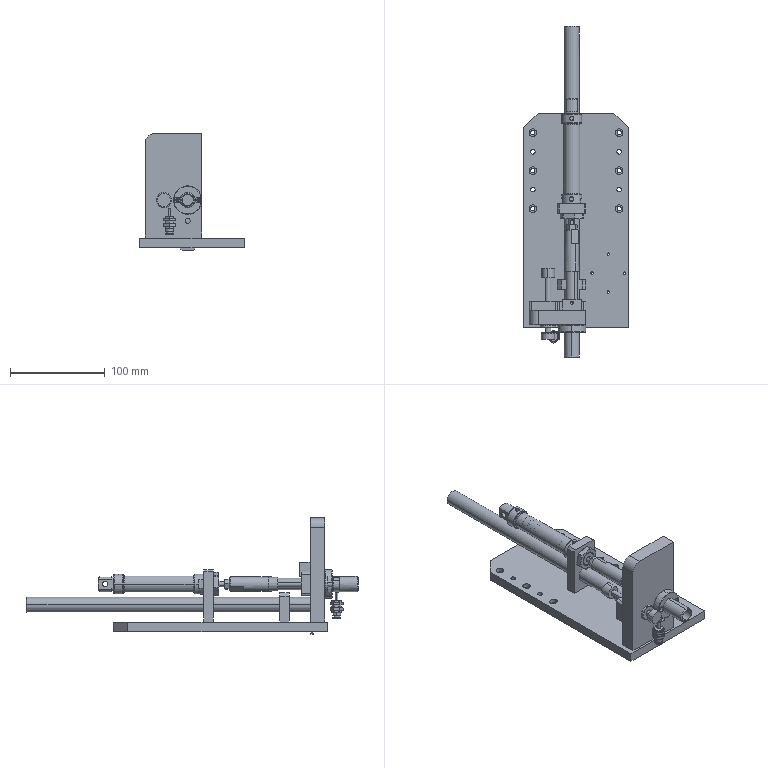Assembly | SolidWorks | mm | 21 component files | 21 solids | 613 faces | box 110 x 349.9 x 123 mm | volume 442250 mm3 | cylinder 275 | plane 190 | cone 140 | spline 8 | commonest cylinder face diameters 6 x30 8 x30 4.5 x30 3.3 x26 12 x17 5 x16 2.5 x16 16 x14
Bill of materials:
gbgb16 MA NutF8 | 1 |  | Thin, flat hexagonal ring with a large central through-bore. One face is chamfered at the corners, and the other face has a thin raised circular collar. The overall shape matches a low-profile hex nut (jam/lock-nut style).
GbgbGuidePlate120F8 | 1 |  | Flat rectangular plate with rounded corners and a stepped top edge (one end taller than the other, joined by a concave fillet). It has four through holes: two small holes near the tall end, one medium hole, and one large hole near the short end.
GbgbLowerMagnetGuideTubeF8 | 1 |  | Hollow flanged bushing: a cylindrical tube with a round flange near one end and a short spigot sticking out past the flange. There is a through bore along the axis, and the flange has two through holes on opposite sides.
GbgbLowerMagnetPushRodF8 | 1 |  | Stepped solid cylindrical pin with a smaller-diameter section and a larger-diameter section. The larger section has a flat cut on its side near the end.
GbgbLowerMagnetTubeFixingSeatF8 | 1 |  | Square block of constant thickness with two chamfered top corners. It has a large round through hole off-centre toward the top, and a small cross hole in one side face.
gbgb1 | 1 |  | Stepped shaft or pin: a long cylindrical middle section with a larger collar near each end, and each collar has a small radial hole. One end is a plain reduced-diameter stub with a hole along its axis. The other end has flat sides and a cross hole through it.
gbgb2 | 1 |  | Long slender rod with a larger cylindrical head at one end. The head has several circumferential grooves. There is a small flat or notch on the shank near the far end.
gbgb4 | 1 |  | Hexagonal nut-like part: a hex prism with a central round through hole and curved chamfers on both faces.
GbgbMagnetBlockFeederF8 | 1 |  | L-shaped bracket made of a thin tall plate with a thicker block at the top. The plate has one round through hole and chamfered lower corners. The block has a small hole on its top face.
GbgbMagnetF8 | 1 |  | Solid round disc with flat parallel faces and small edge chamfers.
GbgbMagnetPlacementTubeF8 | 1 |  | Long, thin-walled straight tube with a constant round cross-section. There is a small rectangular patch partway along its length.
GbgbMagnetPressingHead1F8 | 1 |  | Headed pin: a straight solid cylindrical shank with a larger round head at one end.
GbgbMagnetSleeveSeatF8 | 1 |  | Rectangular plate of constant thickness with two small chamfered top corners. It has two large round through holes in a vertical line and a small cross hole in one side face.
GbgbSleeve | 1 |  | Flanged hollow cylinder (bushing-like): a cylindrical body with a coaxial through bore and a wider, thin circular flange at one end; outer edges are chamfered.
GbgbSpringPostFixingBlockF8 | 1 |  | Plain thick-walled cylindrical sleeve (spacer-like): a solid cylinder with a single coaxial through hole and flat ends, with no visible chamfers or other features.
GbgbSupportPlateF8 | 1 |  | Rectangular flat plate (block) with one rounded corner and a group of holes in its lower half: two larger round holes side by side, two very small holes beside them, and one medium hole below.
GbgbYAxisConnectionPlate | 1 | AL6061 | Elongated flat rectangular plate with two chamfered corners at one end and many round holes, plus one rectangular slot near the opposite end.
Mates:
1. coincident | GbgbYAxisConnectionPlate-1 face at (84.946, 484.94, 390.232) dir (0, 0, 1) | GbgbLowerMagnetTubeFixingSeatF8-1 face at (65.446, 419.94, 390.232) dir (0, 0, -1)
2. concentric | GbgbMagnetPlacementTubeF8-1 face at (80.446, 387.34, 408.232) dir (0, 1, 0) r 8 | GbgbMagnetF8-1 face at (80.446, 384.34, 408.232) dir (0, 1, 0) r 6
3. concentric | GbgbMagnetPressingHead1F8-1 face at (55.446, 364.092, 430.232) dir (0, 1, 0) r 3 | GbgbSpringPostFixingBlockF8-1 face at (55.446, 422.092, 430.232) dir (0, 1, 0) r 7
4. coincident | GbgbYAxisConnectionPlate-1 face at (84.946, 484.94, 390.232) dir (0, 0, 1) | GbgbSupportPlateF8-1 face at (35.446, 387.44, 390.232) dir (0, 0, -1)
5. coincident | GbgbSupportPlateF8-1 face at (65.446, 384.34, 445.232) dir (0, 1, 0) | GbgbMagnetBlockFeederF8-1 face at (80.446, 384.34, 412.732) dir (0, -1, 0)
6. concentric | GbgbMagnetPressingHead1F8-1 face at (55.446, 364.092, 430.232) dir (0, 1, 0) r 3 | GbgbSupportPlateF8-1 face at (55.446, 372.44, 430.232) dir (0, 1, 0) r 6
7. coincident | GbgbSupportPlateF8-1 face at (65.446, 372.44, 445.232) dir (0, -1, 0) | GbgbLowerMagnetGuideTubeF8-1 face at (65.446, 372.44, 430.232) dir (0, 1, 0)
8. coincident | GbgbSupportPlateF8-1 face at (65.446, 387.44, 445.232) dir (0, 1, 0) | GbgbGuidePlate120F8-1 face at (65.446, 387.44, 430.232) dir (0, -1, 0)
9. concentric | GbgbSupportPlateF8-1 face at (80.446, 372.44, 430.232) dir (0, 1, 0) r 6 | GbgbGuidePlate120F8-1 face at (80.446, 387.44, 430.232) dir (0, 1, 0) r 6
10. coincident | GbgbSupportPlateF8-1 face at (90.446, 384.34, 390.232) dir (-1, 0, 0) | GbgbMagnetBlockFeederF8-1 edge at (90.446, 387.34, 438.232) dir (0, 0, -1)
11. parallel | GbgbSupportPlateF8-1 face at (35.446, 387.44, 390.232) dir (-1, 0, 0) | GbgbGuidePlate120F8-1 face at (35.446, 397.44, 442.732) dir (-1, 0, 0)
12. concentric | GbgbGuidePlate120F8-1 face at (80.446, 387.44, 430.232) dir (0, 1, 0) r 6 | GbgbLowerMagnetPushRodF8-1 face at (80.446, 369.237, 430.232) dir (0, -1, 0) r 6
13. coincident | GbgbYAxisConnectionPlate-1 face at (84.946, 484.94, 390.232) dir (0, 0, 1) | GbgbMagnetSleeveSeatF8-4 face at (65.446, 499.94, 390.232) dir (0, 0, -1)
14. coincident | gbgb16 MA NutF8-1 face at (90.67, 489.94, 433.387) dir (0, 1, 0) | GbgbMagnetSleeveSeatF8-4 face at (80.446, 489.94, 417.732) dir (0, -1, 0)
15. concentric | GbgbSupportPlateF8-1 face at (80.446, 375.44, 430.232) dir (0, -1, 0) r 7.5 | GbgbLowerMagnetGuideTubeF8-1 face at (80.446, 385.965, 430.232) dir (0, 1, 0) r 8
16. concentric | GbgbSupportPlateF8-1 face at (69.446, 372.44, 430.232) dir (0, -1, 0) r 1.25 | GbgbLowerMagnetGuideTubeF8-1 face at (69.446, 364.44, 430.232) dir (0, -1, 0) r 1.7
17. coincident | GbgbMagnetPlacementTubeF8-1 face at (80.446, 387.34, 408.232) dir (0, -1, 0) | GbgbMagnetBlockFeederF8-1 face at (80.446, 387.34, 412.732) dir (0, 1, 0)
18. distance | GbgbYAxisConnectionPlate-1 face at (69.946, 388.84, 390.232) dir (1, 0, 0) | GbgbSupportPlateF8-1 face at (70.446, 384.34, 390.232) dir (1, 0, 0)
19. distance | GbgbYAxisConnectionPlate-1 face at (69.946, 383.84, 390.232) dir (0, 1, 0) | GbgbSupportPlateF8-1 face at (65.446, 384.34, 445.232) dir (0, 1, 0)
20. concentric | GbgbMagnetPlacementTubeF8-1 face at (80.446, 387.34, 408.232) dir (0, 1, 0) r 8 | GbgbMagnetSleeveSeatF8-4 face at (80.446, 487.94, 408.232) dir (0, 1, 0) r 8
21. concentric | GbgbYAxisConnectionPlate-1 face at (70.446, 414.94, 380.232) dir (0, 0, -1) r 2.25 | GbgbLowerMagnetTubeFixingSeatF8-1 face at (70.446, 414.94, 390.232) dir (0, 0, -1) r 1.65
22. concentric | GbgbYAxisConnectionPlate-1 face at (90.446, 414.94, 380.232) dir (0, 0, -1) r 2.25 | GbgbLowerMagnetTubeFixingSeatF8-1 face at (90.446, 414.94, 390.232) dir (0, 0, -1) r 1.65
23. concentric | GbgbYAxisConnectionPlate-1 face at (70.446, 494.94, 380.232) dir (0, 0, -1) r 4 | GbgbMagnetSleeveSeatF8-4 face at (70.446, 494.94, 390.232) dir (0, 0, -1) r 1.65
24. concentric | GbgbYAxisConnectionPlate-1 face at (90.446, 494.94, 380.232) dir (0, 0, -1) r 4 | GbgbMagnetSleeveSeatF8-4 face at (90.446, 494.94, 390.232) dir (0, 0, -1) r 1.65
25. coincident | GbgbMagnetF8-1 face at (80.446, 384.34, 408.232) dir (0, -1, 0) | GbgbSupportPlateF8-1 face at (65.446, 384.34, 445.232) dir (0, 1, 0)
26. coincident | GbgbMagnetPressingHead1F8-1 face at (55.446, 422.092, 430.232) dir (0, 1, 0) | GbgbSpringPostFixingBlockF8-1 face at (55.446, 422.092, 430.232) dir (0, -1, 0)
27. concentric | GbgbMagnetPressingHead1F8-1 face at (55.446, 364.092, 430.232) dir (0, 1, 0) r 3 | GbgbSleeve-1 face at (55.446, 387.44, 430.232) dir (0, -1, 0) r 6
28. coincident | GbgbSupportPlateF8-1 face at (65.446, 372.44, 445.232) dir (0, -1, 0) | GbgbSleeve-1 face at (55.446, 372.44, 430.232) dir (0, 1, 0)
29. concentric | gbgbMA16x35SCA_0_+-2/gbgb1-1 face at (80.446, 492.4, 430.232) dir (0, 1, 0) r 7.188 | GbgbMagnetSleeveSeatF8-4 face at (80.446, 499.94, 430.232) dir (0, 1, 0) r 7.25
30. coincident | GbgbLowerMagnetPushRodF8-1 face at (74.05, 472.93, 434.148) dir (0, 1, 0) | gbgbMA16x35SCA_0_+-2/gbgb4-1 face at (81.97, 472.93, 432.214) dir (0, -1, 0)
31. coincident | gbgbMA16x35SCA_0_+-2/gbgb1-1 face at (80.446, 499.94, 439.282) dir (0, -1, 0) | GbgbMagnetSleeveSeatF8-4 face at (80.446, 499.94, 417.732) dir (0, 1, 0)
32. parallel | gbgbMA16x35SCA_0_+-2/gbgb1-1 face at (89.946, 499.94, 440.732) dir (1, 0, 0) | GbgbMagnetSleeveSeatF8-4 face at (95.446, 499.94, 390.232) dir (1, 0, 0)
33. distance | GbgbMagnetBlockFeederF8-1 face at (80.446, 384.34, 448.232) dir (0, 0, 1) | GbgbSupportPlateF8-1 face at (70.446, 384.34, 470.232) dir (0, 0, -1)
34. parallel | GbgbMagnetPlacementTubeF8-1 face at (87.946, 499.84, 413.232) dir (1, 0, 0) | GbgbMagnetSleeveSeatF8-4 face at (95.446, 499.94, 390.232) dir (1, 0, 0)
35. distance | GbgbMagnetPressingHead1F8-1 face at (55.446, 364.092, 430.232) dir (0, 1, 0) | GbgbSleeve-1 face at (55.446, 369.44, 430.232) dir (0, -1, 0)
36. coincident | gbgbCJPB6-5_BODYF8-1 axis at (-80.9, 0, 0) dir (1, 0, 0) | gbgbCJPB6-5-B_RODF8-1 axis at (80.9, 0, 0) dir (-1, 0, 0)
37. angle | gbgbCJPB6-5-B_RODF8-1 plane at (0, 0, 0) dir (0, 0, -1) | gbgbCJPB6-5_BODYF8-1 plane at (0, 0, 0) dir (0, 0, -1)
38. coincident | gbgbCJPB6-5_BODYF8-1 axis at (80.9, 0, 0) dir (-1, 0, 0) | gbgbSNPS-006_CJPF8-1 axis at (-79.4, 0, 0) dir (1, 0, 0)
39. distance | gbgbSNPS-006_CJPF8-2 plane at (7.5, 0, 0) dir (-1, 0, 0) | gbgbCJPB6-5_BODYF8-1 plane at (0, 0, 0) dir (1, 0, 0)
40. coincident | gbgbCJPB6-5_BODYF8-1 axis at (80.9, 0, 0) dir (-1, 0, 0) | gbgbSNPS-006_CJPF8-2 axis at (-73.4, 0, 0) dir (1, 0, 0)
41. angle | gbgbSNPS-006_CJPF8-2 plane at (7.5, 0, 0) dir (0, 0, -1) | gbgbCJPB6-5_BODYF8-1 plane at (0, 0, 0) dir (0, 0, -1)
42. concentric | gbgb1-1 face at (-17.54, 0, 0) dir (1, 0, 0) r 7.188 | gbgb2-1 face at (-1.203, 0, 0) dir (1, 0, 0) r 3
43. concentric | gbgb2-1 face at (-1.203, 0, 0) dir (1, 0, 0) r 3 | gbgb4-1 face at (-34.51, 0, 0) dir (-1, 0, 0) r 3
44. coincident | gbgb2-1 edge at (-32.01, -1.922, -2.303) dir (0, -0.2856, 0.9584) | gbgb4-1 face at (-32.01, 1.982, 1.523) dir (1, 0, 0)
45. distance | gbgb1-1 face at (65, 4, 0) dir (-1, 0, 0) | gbgb2-1 face at (64.99, -1.078, 3.618) dir (1, 0, 0)